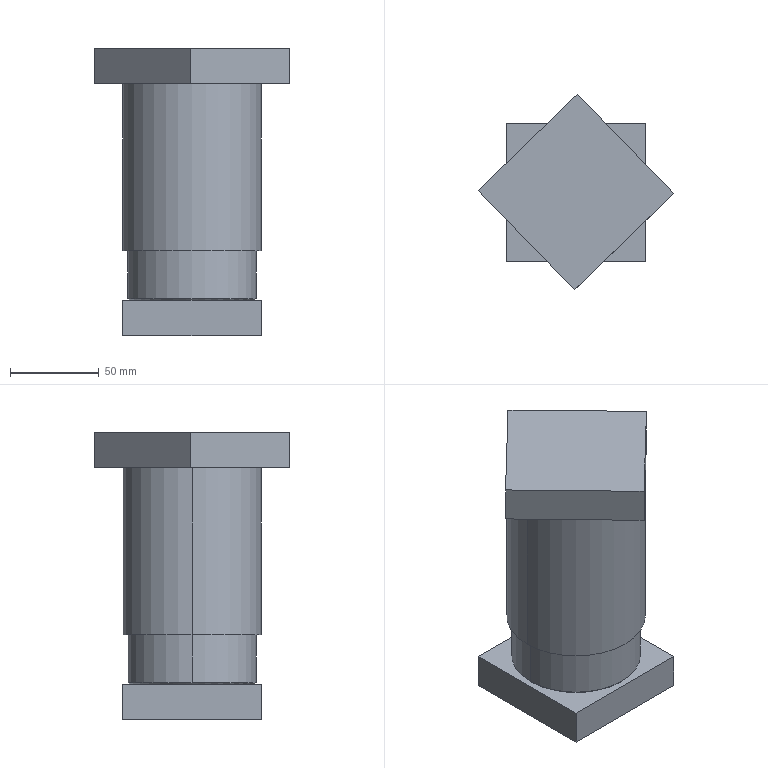CAM job | Mastercam | mm | 11 operations | part box 110.29 x 110.29 x 162
1. Drill/Counterbore | 6 - 6 倒角刀
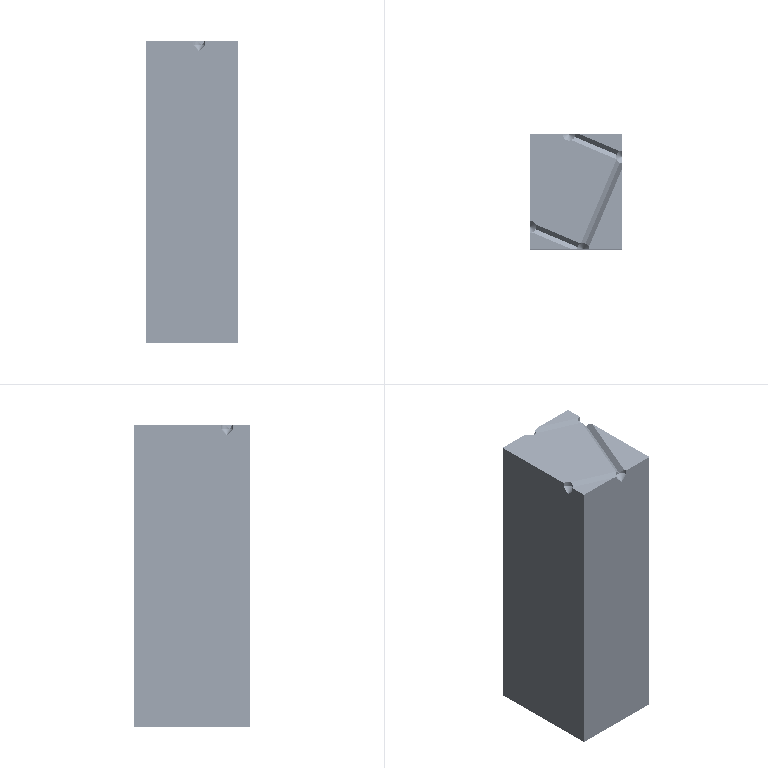2. Drill/Counterbore | 6 - 6 倒角刀
3. Peck Drill | 19 - 5 钻头
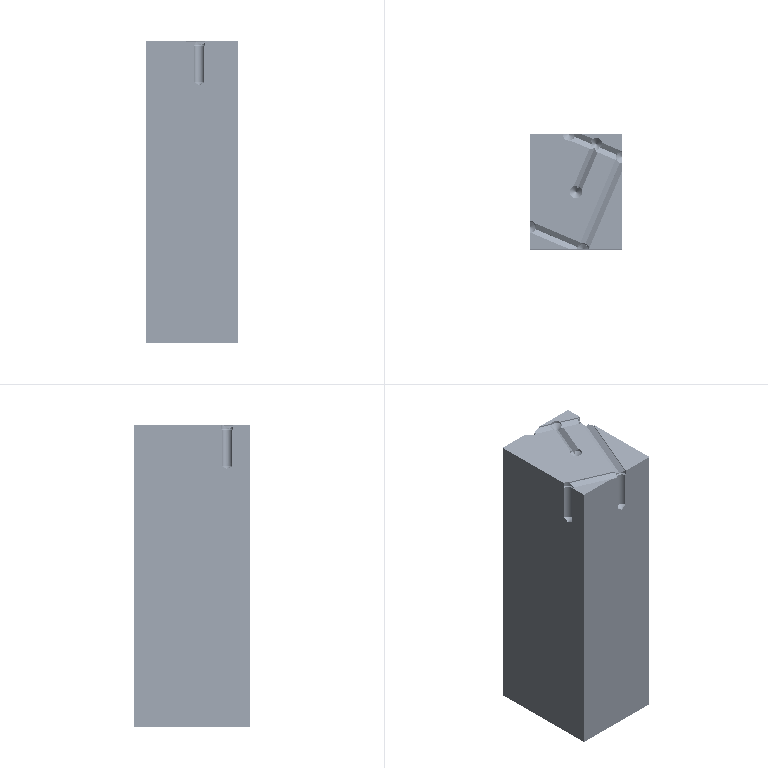4. Drill/Counterbore | 6 - 6 倒角刀
5. Contour (Ramp) | 4 - 6 平铣刀
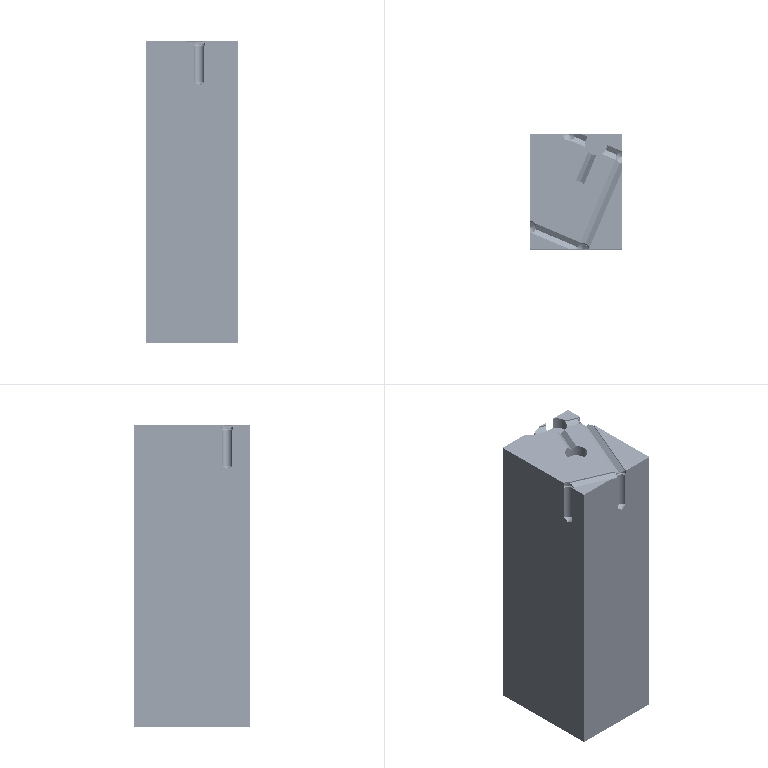6. Contour (2D) | 5 - 6 平铣刀
7. Chamfer Drill | 6 - 6 倒角刀
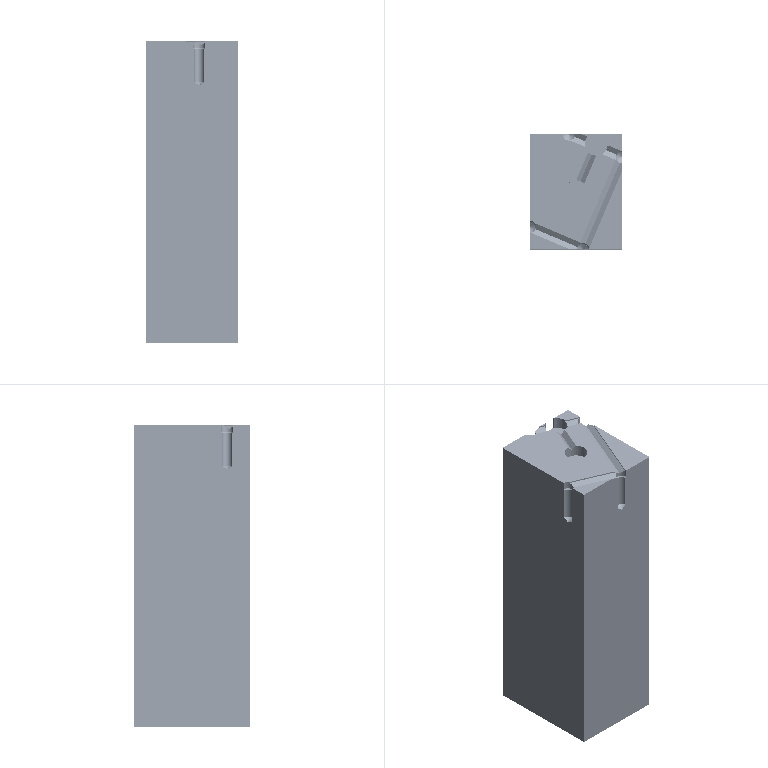8. Model Chamfer | 6 - 6 倒角刀
9. Contour (Ramp) | 4 - 6 平铣刀
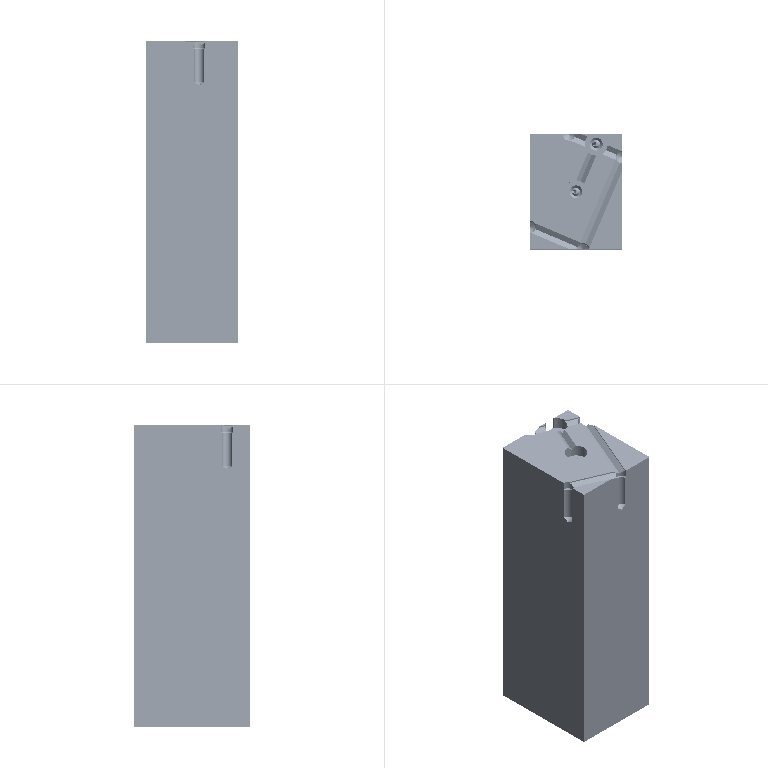10. Contour (2D) | 5 - 6 平铣刀
11. Contour (2D chamfer) | 6 - 6 倒角刀